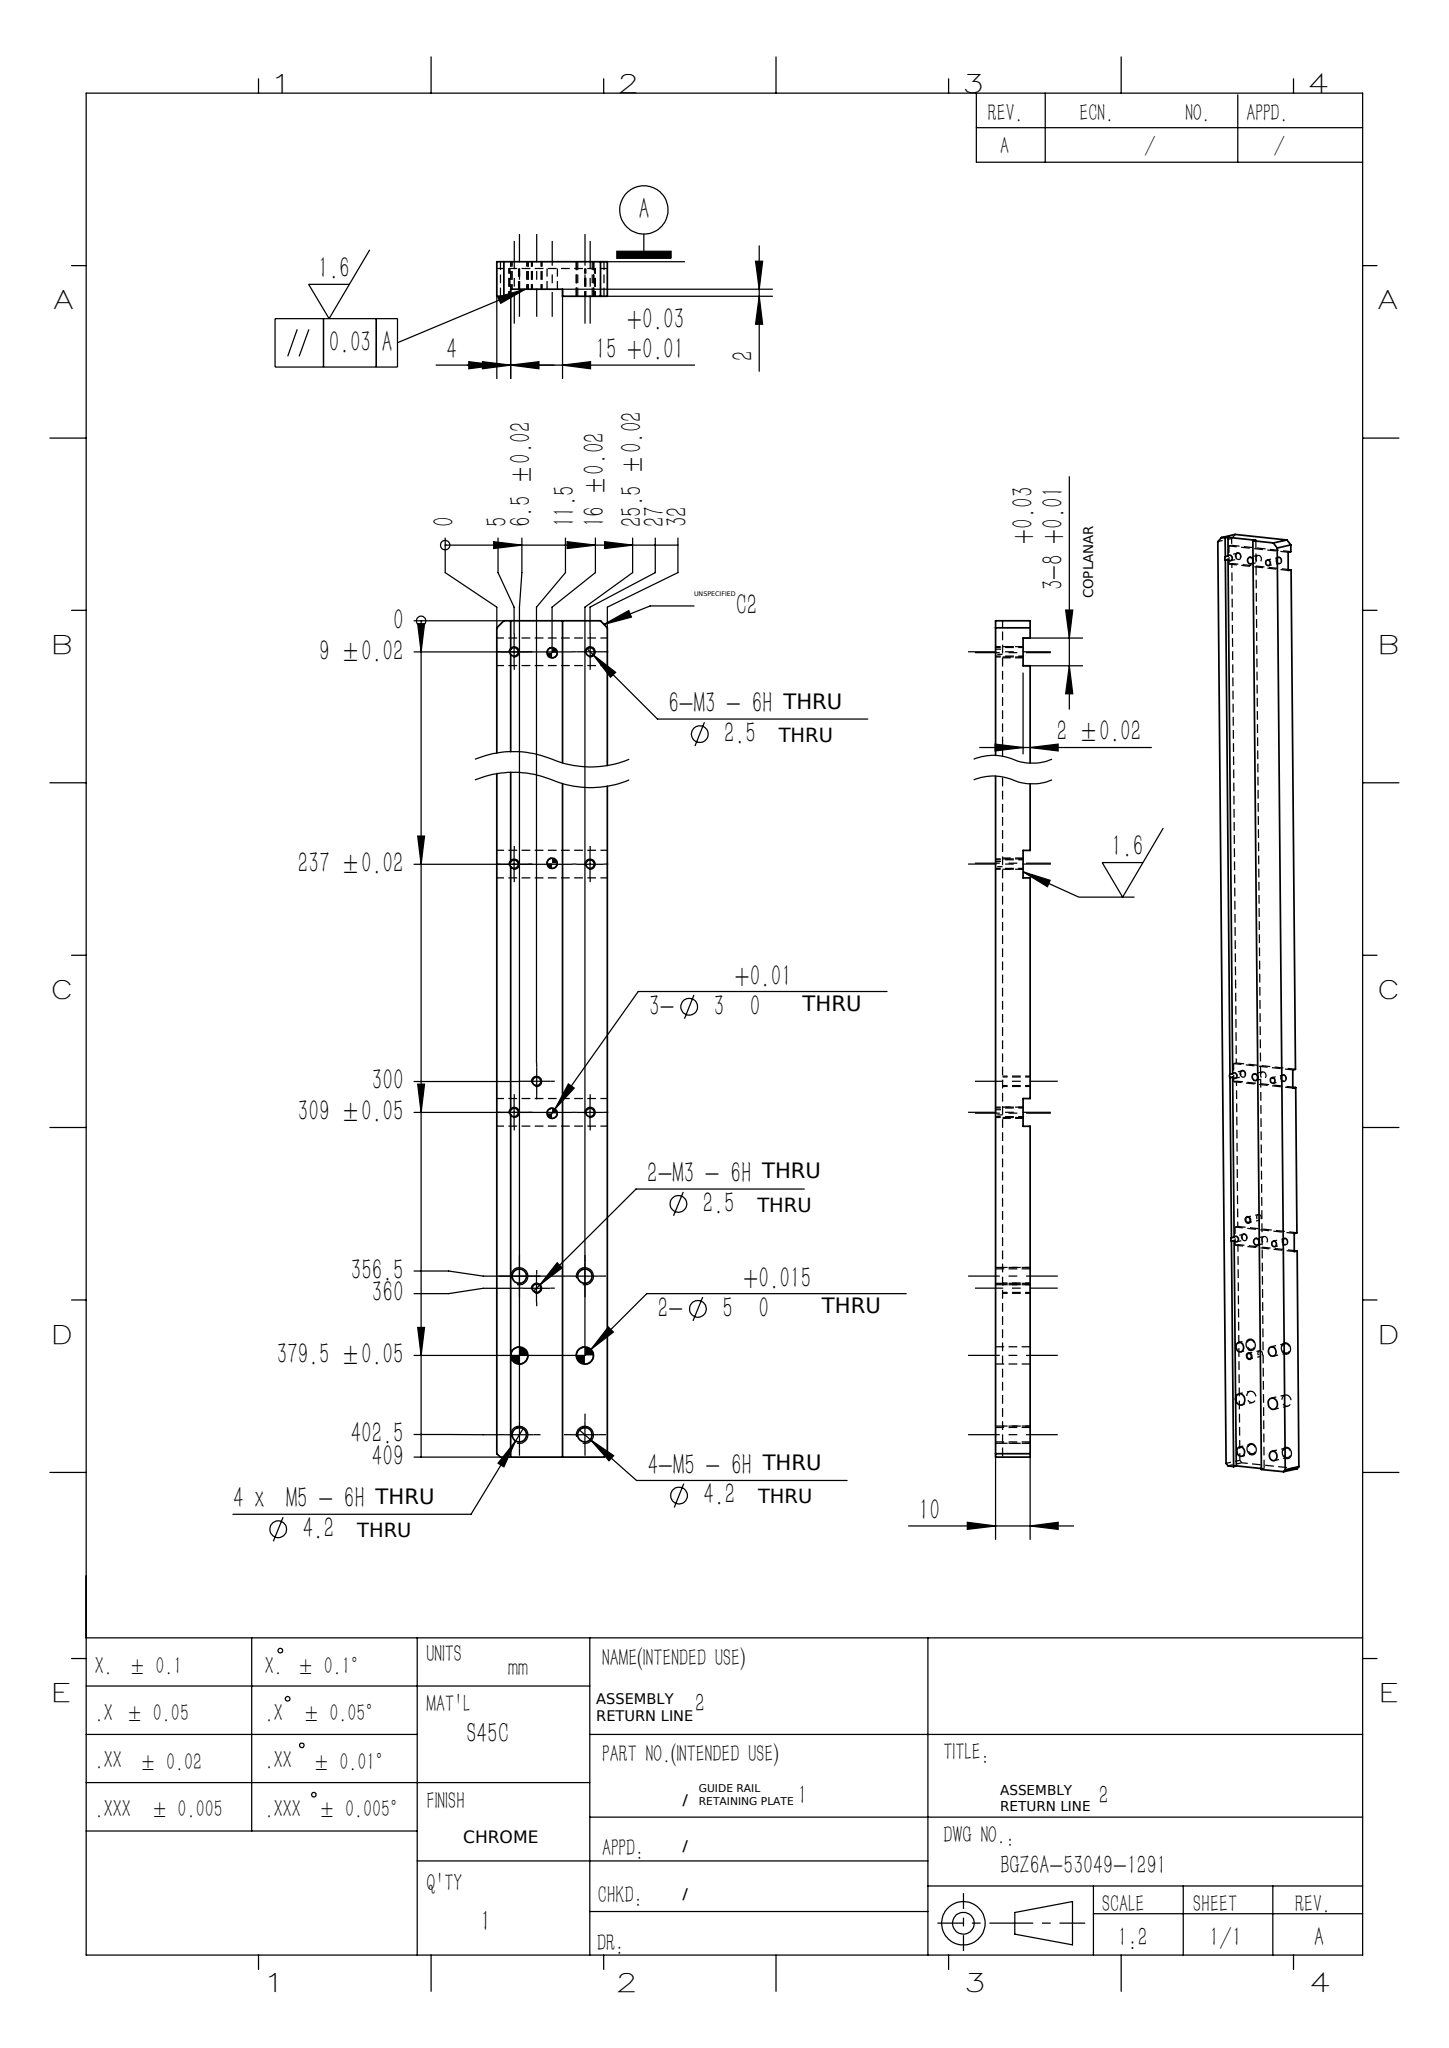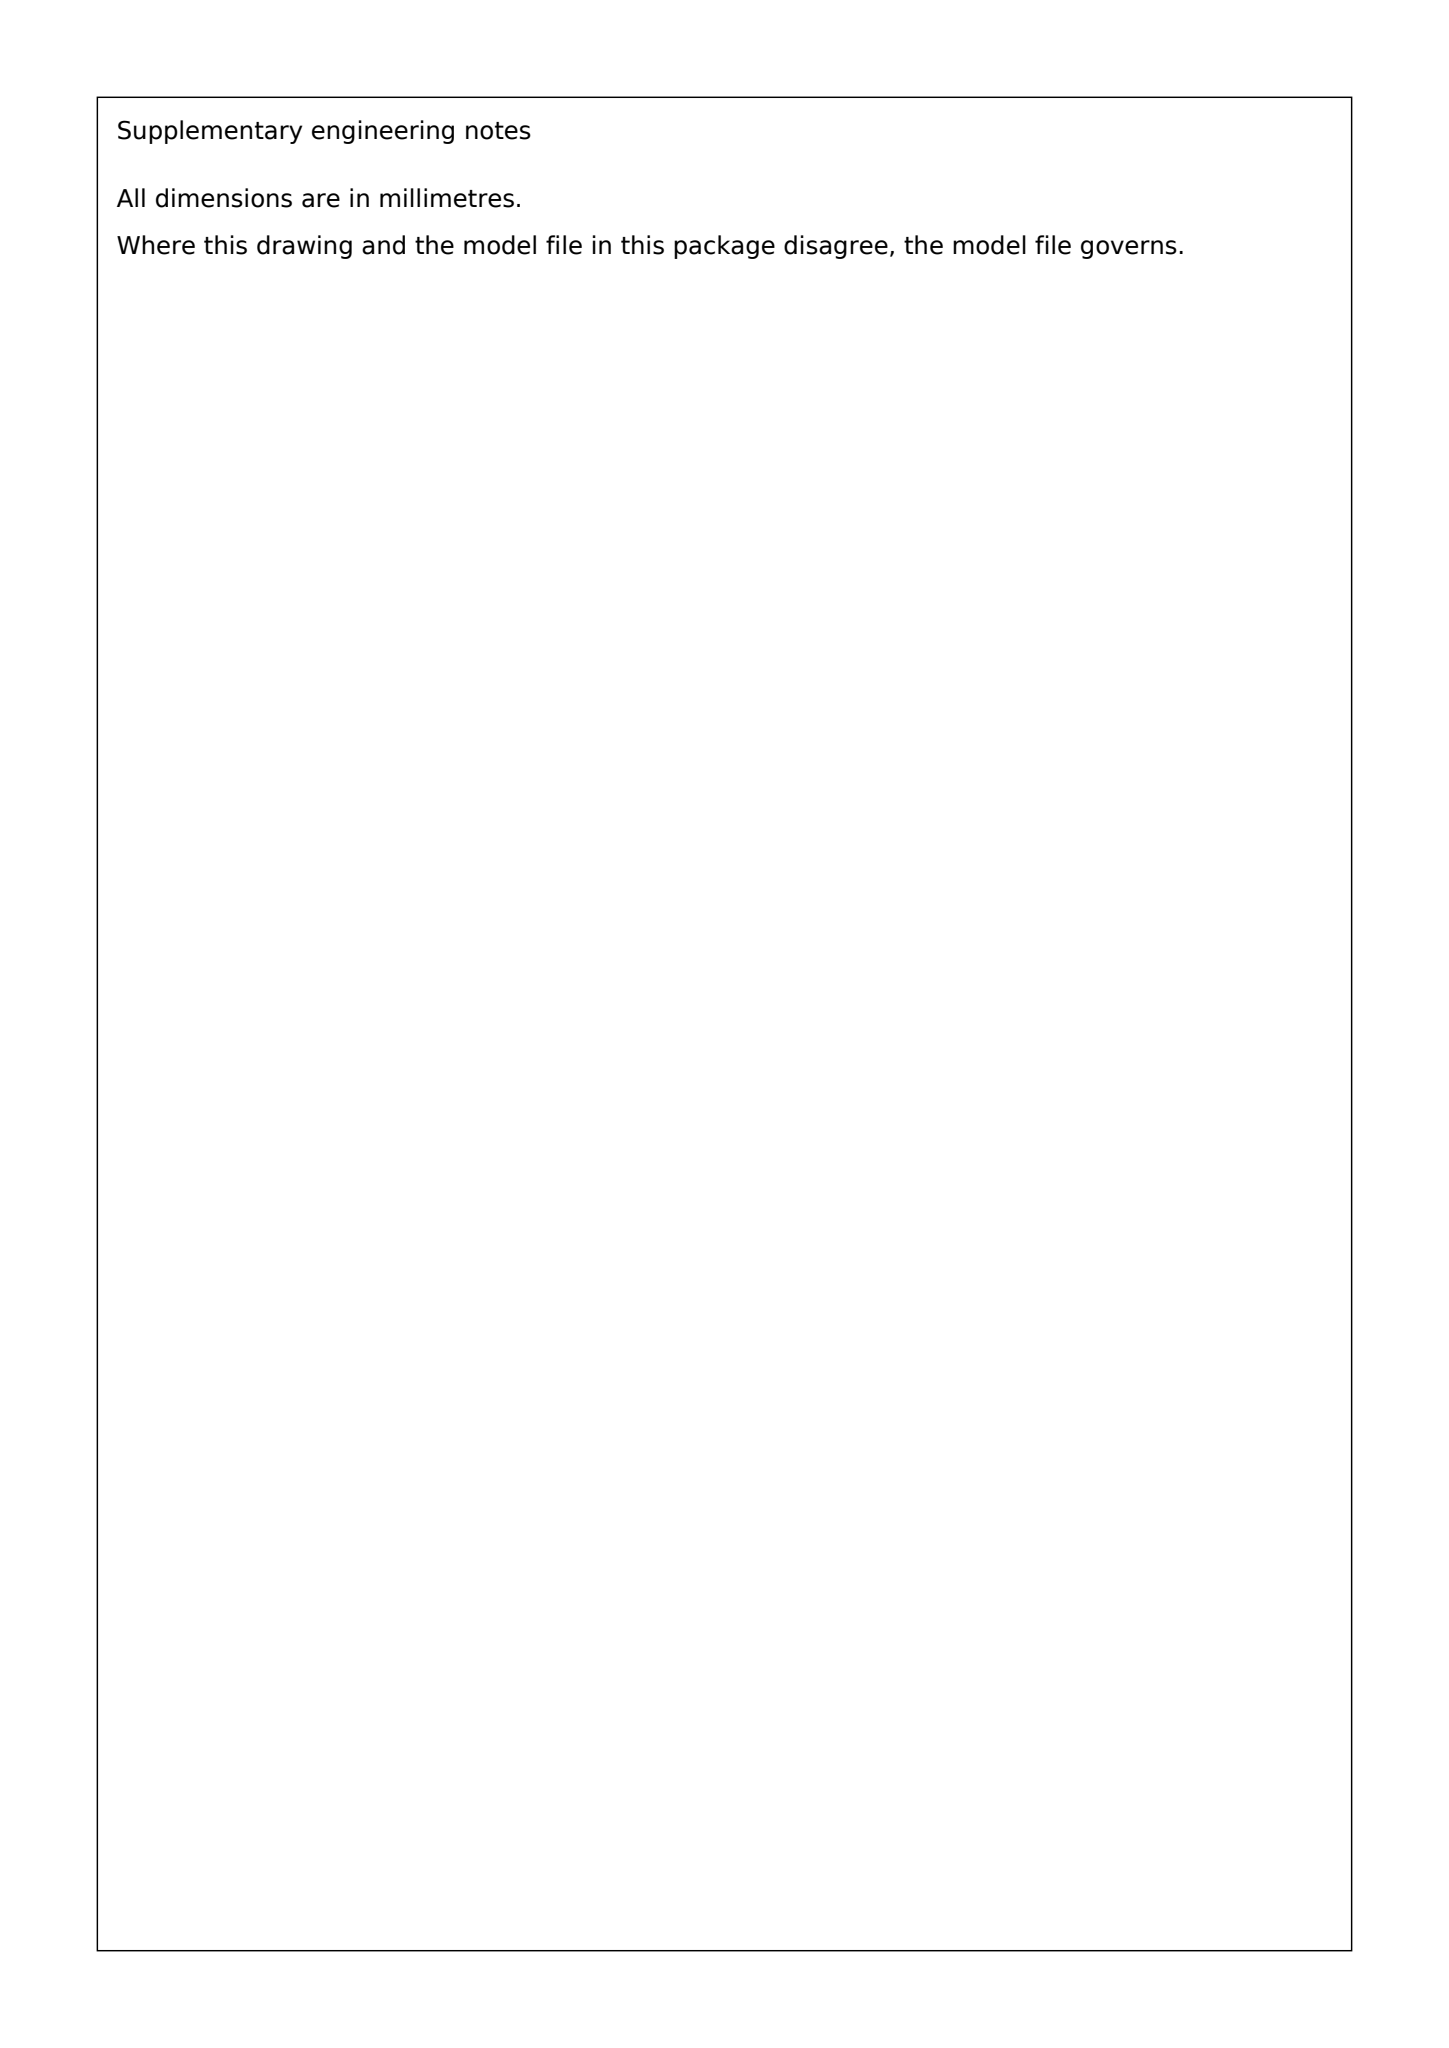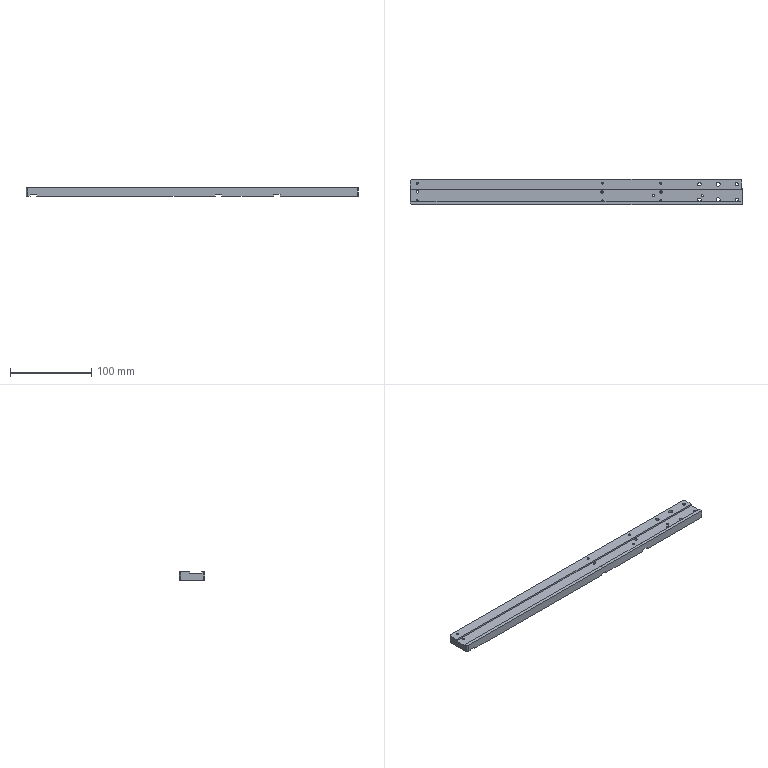Part | SolidWorks | mm | 1 solid | 63 faces | box 409 x 32 x 10 mm | volume 115758 mm3 | cylinder 34 | plane 29 | commonest cylinder face diameters 2.5 x16 4.2 x8 3 x6 5 x4